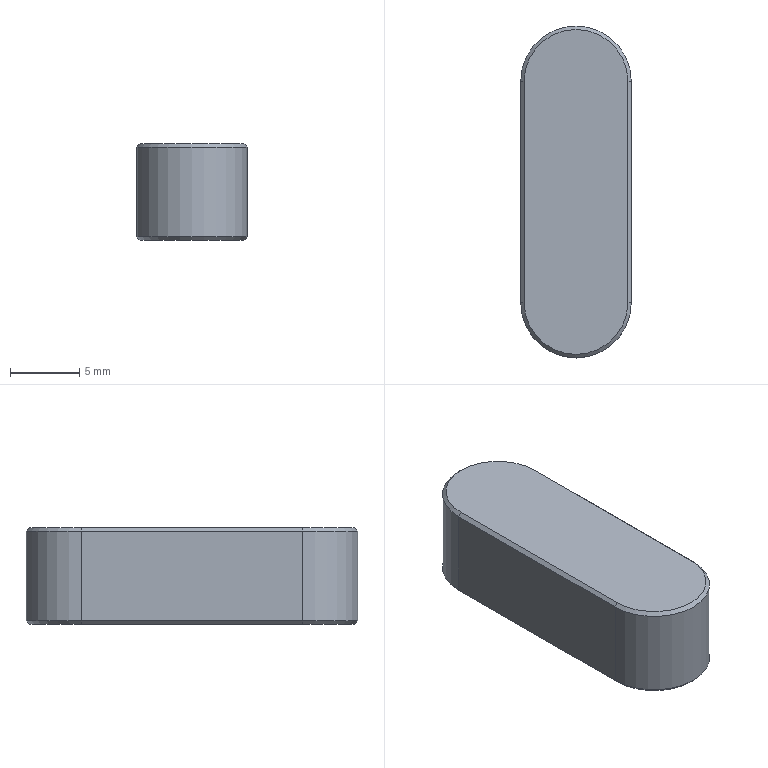Component | NX | KEY_A_8X7X24 | 1 solid | 14 faces | box 8 x 24 x 7 mm | volume 1244 mm3 | plane 8 | cone 4 | cylinder 2 | commonest cylinder face diameters 8 x2
STEP:
#1=CARTESIAN_POINT('',(0.,0.,0.));
#2=DIRECTION('',(0.,0.,1.));
#3=DIRECTION('',(1.,0.,0.));
#4=AXIS2_PLACEMENT_3D('',#1,#2,#3);
#5=CARTESIAN_POINT('',(375.053,-142.75,-118.));
#6=VERTEX_POINT('',#5);
#7=CARTESIAN_POINT('',(375.053,-158.75,-118.));
#8=VERTEX_POINT('',#7);
#9=CARTESIAN_POINT('',(375.053,-150.75,-118.));
#10=DIRECTION('',(0.,-1.,0.));
#11=VECTOR('',#10,1.);
#12=LINE('',#9,#11);
#13=CARTESIAN_POINT('',(378.803,-150.75,-118.));
#14=DIRECTION('',(0.,0.,1.));
#15=DIRECTION('',(1.,0.,0.));
#16=AXIS2_PLACEMENT_3D('',#13,#14,#15);
#17=PLANE('',#16);
#18=CARTESIAN_POINT('',(-3.75,0.));
#19=DIRECTION('',(0.,-1.));
#20=VECTOR('',#19,1.);
#21=LINE('',#18,#20);
#22=(GEOMETRIC_REPRESENTATION_CONTEXT(2)PARAMETRIC_REPRESENTATION_CONTEXT()REPRESENTATION_CONTEXT('',''));
#23=DEFINITIONAL_REPRESENTATION('',(#21),#22);
#24=PCURVE('',#17,#23);
#25=CARTESIAN_POINT('',(374.803,-150.75,-118.25));
#26=DIRECTION('',(0.7071,0.,-0.7071));
#27=DIRECTION('',(0.,1.,0.));
#28=AXIS2_PLACEMENT_3D('',#25,#26,#27);
#29=PLANE('',#28);
#30=CARTESIAN_POINT('',(0.,0.3536));
#31=DIRECTION('',(-1.,0.));
#32=VECTOR('',#31,1.);
#33=LINE('',#30,#32);
#34=(GEOMETRIC_REPRESENTATION_CONTEXT(2)PARAMETRIC_REPRESENTATION_CONTEXT()REPRESENTATION_CONTEXT('',''));
#35=DEFINITIONAL_REPRESENTATION('',(#33),#34);
#36=PCURVE('',#29,#35);
#37=SURFACE_CURVE('',#12,(#24,#36),.PCURVE_S1.);
#38=EDGE_CURVE('',#6,#8,#37,.T.);
#39=ORIENTED_EDGE('',*,*,#38,.T.);
#40=CARTESIAN_POINT('',(382.553,-158.75,-118.));
#41=VERTEX_POINT('',#40);
#42=CARTESIAN_POINT('',(378.803,-158.75,-118.));
#43=DIRECTION('',(0.,0.,1.));
#44=DIRECTION('',(1.,0.,0.));
#45=AXIS2_PLACEMENT_3D('',#42,#43,#44);
#46=CIRCLE('',#45,3.75);
#47=CARTESIAN_POINT('',(0.,-8.));
#48=DIRECTION('',(1.,0.));
#49=AXIS2_PLACEMENT_2D('',#47,#48);
#50=CIRCLE('',#49,3.75);
#51=(GEOMETRIC_REPRESENTATION_CONTEXT(2)PARAMETRIC_REPRESENTATION_CONTEXT()REPRESENTATION_CONTEXT('',''));
#52=DEFINITIONAL_REPRESENTATION('',(#50),#51);
#53=PCURVE('',#17,#52);
#54=CARTESIAN_POINT('',(378.803,-158.75,-118.));
#55=DIRECTION('',(0.,0.,-1.));
#56=DIRECTION('',(-1.,0.,0.));
#57=AXIS2_PLACEMENT_3D('',#54,#55,#56);
#58=CONICAL_SURFACE('',#57,3.75,0.7854);
#59=CARTESIAN_POINT('',(9.425,0.));
#60=DIRECTION('',(-1.,0.));
#61=VECTOR('',#60,1.);
#62=LINE('',#59,#61);
#63=(GEOMETRIC_REPRESENTATION_CONTEXT(2)PARAMETRIC_REPRESENTATION_CONTEXT()REPRESENTATION_CONTEXT('',''));
#64=DEFINITIONAL_REPRESENTATION('',(#62),#63);
#65=PCURVE('',#58,#64);
#66=SURFACE_CURVE('',#46,(#53,#65),.PCURVE_S1.);
#67=EDGE_CURVE('',#8,#41,#66,.T.);
#68=ORIENTED_EDGE('',*,*,#67,.T.);
#69=CARTESIAN_POINT('',(382.553,-142.75,-118.));
#70=VERTEX_POINT('',#69);
#71=CARTESIAN_POINT('',(382.553,-150.75,-118.));
#72=DIRECTION('',(0.,1.,0.));
#73=VECTOR('',#72,1.);
#74=LINE('',#71,#73);
#75=CARTESIAN_POINT('',(3.75,0.));
#76=DIRECTION('',(0.,1.));
#77=VECTOR('',#76,1.);
#78=LINE('',#75,#77);
#79=(GEOMETRIC_REPRESENTATION_CONTEXT(2)PARAMETRIC_REPRESENTATION_CONTEXT()REPRESENTATION_CONTEXT('',''));
#80=DEFINITIONAL_REPRESENTATION('',(#78),#79);
#81=PCURVE('',#17,#80);
#82=CARTESIAN_POINT('',(382.803,-150.75,-118.25));
#83=DIRECTION('',(-0.7071,0.,-0.7071));
#84=DIRECTION('',(0.,-1.,0.));
#85=AXIS2_PLACEMENT_3D('',#82,#83,#84);
#86=PLANE('',#85);
#87=CARTESIAN_POINT('',(0.,0.3536));
#88=DIRECTION('',(-1.,0.));
#89=VECTOR('',#88,1.);
#90=LINE('',#87,#89);
#91=(GEOMETRIC_REPRESENTATION_CONTEXT(2)PARAMETRIC_REPRESENTATION_CONTEXT()REPRESENTATION_CONTEXT('',''));
#92=DEFINITIONAL_REPRESENTATION('',(#90),#91);
#93=PCURVE('',#86,#92);
#94=SURFACE_CURVE('',#74,(#81,#93),.PCURVE_S1.);
#95=EDGE_CURVE('',#41,#70,#94,.T.);
#96=ORIENTED_EDGE('',*,*,#95,.T.);
#97=CARTESIAN_POINT('',(378.803,-142.75,-118.));
#98=DIRECTION('',(0.,0.,1.));
#99=DIRECTION('',(1.,0.,0.));
#100=AXIS2_PLACEMENT_3D('',#97,#98,#99);
#101=CIRCLE('',#100,3.75);
#102=CARTESIAN_POINT('',(0.,8.));
#103=DIRECTION('',(1.,0.));
#104=AXIS2_PLACEMENT_2D('',#102,#103);
#105=CIRCLE('',#104,3.75);
#106=(GEOMETRIC_REPRESENTATION_CONTEXT(2)PARAMETRIC_REPRESENTATION_CONTEXT()REPRESENTATION_CONTEXT('',''));
#107=DEFINITIONAL_REPRESENTATION('',(#105),#106);
#108=PCURVE('',#17,#107);
#109=CARTESIAN_POINT('',(378.803,-142.75,-118.));
#110=DIRECTION('',(0.,0.,-1.));
#111=DIRECTION('',(-1.,0.,0.));
#112=AXIS2_PLACEMENT_3D('',#109,#110,#111);
#113=CONICAL_SURFACE('',#112,3.75,0.7854);
#114=CARTESIAN_POINT('',(3.142,0.));
#115=DIRECTION('',(-1.,0.));
#116=VECTOR('',#115,1.);
#117=LINE('',#114,#116);
#118=(GEOMETRIC_REPRESENTATION_CONTEXT(2)PARAMETRIC_REPRESENTATION_CONTEXT()REPRESENTATION_CONTEXT('',''));
#119=DEFINITIONAL_REPRESENTATION('',(#117),#118);
#120=PCURVE('',#113,#119);
#121=SURFACE_CURVE('',#101,(#108,#120),.PCURVE_S1.);
#122=EDGE_CURVE('',#70,#6,#121,.T.);
#123=ORIENTED_EDGE('',*,*,#122,.T.);
#124=EDGE_LOOP('',(#39,#68,#96,#123));
#125=FACE_BOUND('',#124,.T.);
#126=ADVANCED_FACE('',(#125),#17,.T.);
#127=CARTESIAN_POINT('',(374.803,-142.75,-118.25));
#128=VERTEX_POINT('',#127);
#129=CARTESIAN_POINT('',(374.803,-142.75,-124.75));
#130=VERTEX_POINT('',#129);
#131=CARTESIAN_POINT('',(374.803,-142.75,-125.));
#132=DIRECTION('',(0.,0.,-1.));
#133=VECTOR('',#132,1.);
#134=LINE('',#131,#133);
#135=CARTESIAN_POINT('',(374.803,-150.75,-125.));
#136=DIRECTION('',(-1.,0.,0.));
#137=DIRECTION('',(0.,0.,1.));
#138=AXIS2_PLACEMENT_3D('',#135,#136,#137);
#139=PLANE('',#138);
#140=CARTESIAN_POINT('',(0.,8.));
#141=DIRECTION('',(-1.,0.));
#142=VECTOR('',#141,1.);
#143=LINE('',#140,#142);
#144=(GEOMETRIC_REPRESENTATION_CONTEXT(2)PARAMETRIC_REPRESENTATION_CONTEXT()REPRESENTATION_CONTEXT('',''));
#145=DEFINITIONAL_REPRESENTATION('',(#143),#144);
#146=PCURVE('',#139,#145);
#147=CARTESIAN_POINT('',(378.803,-142.75,-125.));
#148=DIRECTION('',(0.,0.,1.));
#149=DIRECTION('',(1.,0.,0.));
#150=AXIS2_PLACEMENT_3D('',#147,#148,#149);
#151=CYLINDRICAL_SURFACE('',#150,4.);
#152=CARTESIAN_POINT('',(3.142,0.));
#153=DIRECTION('',(0.,-1.));
#154=VECTOR('',#153,1.);
#155=LINE('',#152,#154);
#156=(GEOMETRIC_REPRESENTATION_CONTEXT(2)PARAMETRIC_REPRESENTATION_CONTEXT()REPRESENTATION_CONTEXT('',''));
#157=DEFINITIONAL_REPRESENTATION('',(#155),#156);
#158=PCURVE('',#151,#157);
#159=SURFACE_CURVE('',#134,(#146,#158),.PCURVE_S1.);
#160=EDGE_CURVE('',#128,#130,#159,.T.);
#161=ORIENTED_EDGE('',*,*,#160,.T.);
#162=CARTESIAN_POINT('',(374.803,-158.75,-124.75));
#163=VERTEX_POINT('',#162);
#164=CARTESIAN_POINT('',(374.803,-150.75,-124.75));
#165=DIRECTION('',(0.,-1.,0.));
#166=VECTOR('',#165,1.);
#167=LINE('',#164,#166);
#168=CARTESIAN_POINT('',(0.25,0.));
#169=DIRECTION('',(0.,-1.));
#170=VECTOR('',#169,1.);
#171=LINE('',#168,#170);
#172=(GEOMETRIC_REPRESENTATION_CONTEXT(2)PARAMETRIC_REPRESENTATION_CONTEXT()REPRESENTATION_CONTEXT('',''));
#173=DEFINITIONAL_REPRESENTATION('',(#171),#172);
#174=PCURVE('',#139,#173);
#175=CARTESIAN_POINT('',(374.803,-150.75,-124.75));
#176=DIRECTION('',(0.7071,0.,0.7071));
#177=DIRECTION('',(0.,-1.,0.));
#178=AXIS2_PLACEMENT_3D('',#175,#176,#177);
#179=PLANE('',#178);
#180=CARTESIAN_POINT('',(0.,0.));
#181=DIRECTION('',(1.,0.));
#182=VECTOR('',#181,1.);
#183=LINE('',#180,#182);
#184=(GEOMETRIC_REPRESENTATION_CONTEXT(2)PARAMETRIC_REPRESENTATION_CONTEXT()REPRESENTATION_CONTEXT('',''));
#185=DEFINITIONAL_REPRESENTATION('',(#183),#184);
#186=PCURVE('',#179,#185);
#187=SURFACE_CURVE('',#167,(#174,#186),.PCURVE_S1.);
#188=EDGE_CURVE('',#130,#163,#187,.T.);
#189=ORIENTED_EDGE('',*,*,#188,.T.);
#190=CARTESIAN_POINT('',(374.803,-158.75,-118.25));
#191=VERTEX_POINT('',#190);
#192=CARTESIAN_POINT('',(374.803,-158.75,-125.));
#193=DIRECTION('',(0.,0.,1.));
#194=VECTOR('',#193,1.);
#195=LINE('',#192,#194);
#196=CARTESIAN_POINT('',(0.,-8.));
#197=DIRECTION('',(1.,0.));
#198=VECTOR('',#197,1.);
#199=LINE('',#196,#198);
#200=(GEOMETRIC_REPRESENTATION_CONTEXT(2)PARAMETRIC_REPRESENTATION_CONTEXT()REPRESENTATION_CONTEXT('',''));
#201=DEFINITIONAL_REPRESENTATION('',(#199),#200);
#202=PCURVE('',#139,#201);
#203=CARTESIAN_POINT('',(378.803,-158.75,-125.));
#204=DIRECTION('',(0.,0.,1.));
#205=DIRECTION('',(1.,0.,0.));
#206=AXIS2_PLACEMENT_3D('',#203,#204,#205);
#207=CYLINDRICAL_SURFACE('',#206,4.);
#208=CARTESIAN_POINT('',(3.142,0.));
#209=DIRECTION('',(0.,1.));
#210=VECTOR('',#209,1.);
#211=LINE('',#208,#210);
#212=(GEOMETRIC_REPRESENTATION_CONTEXT(2)PARAMETRIC_REPRESENTATION_CONTEXT()REPRESENTATION_CONTEXT('',''));
#213=DEFINITIONAL_REPRESENTATION('',(#211),#212);
#214=PCURVE('',#207,#213);
#215=SURFACE_CURVE('',#195,(#202,#214),.PCURVE_S1.);
#216=EDGE_CURVE('',#163,#191,#215,.T.);
#217=ORIENTED_EDGE('',*,*,#216,.T.);
#218=CARTESIAN_POINT('',(374.803,-150.75,-118.25));
#219=DIRECTION('',(0.,1.,0.));
#220=VECTOR('',#219,1.);
#221=LINE('',#218,#220);
#222=CARTESIAN_POINT('',(6.75,0.));
#223=DIRECTION('',(0.,1.));
#224=VECTOR('',#223,1.);
#225=LINE('',#222,#224);
#226=(GEOMETRIC_REPRESENTATION_CONTEXT(2)PARAMETRIC_REPRESENTATION_CONTEXT()REPRESENTATION_CONTEXT('',''));
#227=DEFINITIONAL_REPRESENTATION('',(#225),#226);
#228=PCURVE('',#139,#227);
#229=CARTESIAN_POINT('',(0.,0.));
#230=DIRECTION('',(1.,0.));
#231=VECTOR('',#230,1.);
#232=LINE('',#229,#231);
#233=(GEOMETRIC_REPRESENTATION_CONTEXT(2)PARAMETRIC_REPRESENTATION_CONTEXT()REPRESENTATION_CONTEXT('',''));
#234=DEFINITIONAL_REPRESENTATION('',(#232),#233);
#235=PCURVE('',#29,#234);
#236=SURFACE_CURVE('',#221,(#228,#235),.PCURVE_S1.);
#237=EDGE_CURVE('',#191,#128,#236,.T.);
#238=ORIENTED_EDGE('',*,*,#237,.T.);
#239=EDGE_LOOP('',(#161,#189,#217,#238));
#240=FACE_BOUND('',#239,.T.);
#241=ADVANCED_FACE('',(#240),#139,.T.);
#242=CARTESIAN_POINT('',(382.553,-142.75,-125.));
#243=VERTEX_POINT('',#242);
#244=CARTESIAN_POINT('',(382.553,-158.75,-125.));
#245=VERTEX_POINT('',#244);
#246=CARTESIAN_POINT('',(382.553,-150.75,-125.));
#247=DIRECTION('',(0.,-1.,0.));
#248=VECTOR('',#247,1.);
#249=LINE('',#246,#248);
#250=CARTESIAN_POINT('',(378.803,-150.75,-125.));
#251=DIRECTION('',(0.,0.,-1.));
#252=DIRECTION('',(-1.,0.,0.));
#253=AXIS2_PLACEMENT_3D('',#250,#251,#252);
#254=PLANE('',#253);
#255=CARTESIAN_POINT('',(-3.75,0.));
#256=DIRECTION('',(0.,-1.));
#257=VECTOR('',#256,1.);
#258=LINE('',#255,#257);
#259=(GEOMETRIC_REPRESENTATION_CONTEXT(2)PARAMETRIC_REPRESENTATION_CONTEXT()REPRESENTATION_CONTEXT('',''));
#260=DEFINITIONAL_REPRESENTATION('',(#258),#259);
#261=PCURVE('',#254,#260);
#262=CARTESIAN_POINT('',(382.803,-150.75,-124.75));
#263=DIRECTION('',(-0.7071,0.,0.7071));
#264=DIRECTION('',(0.,1.,0.));
#265=AXIS2_PLACEMENT_3D('',#262,#263,#264);
#266=PLANE('',#265);
#267=CARTESIAN_POINT('',(0.,0.3536));
#268=DIRECTION('',(-1.,0.));
#269=VECTOR('',#268,1.);
#270=LINE('',#267,#269);
#271=(GEOMETRIC_REPRESENTATION_CONTEXT(2)PARAMETRIC_REPRESENTATION_CONTEXT()REPRESENTATION_CONTEXT('',''));
#272=DEFINITIONAL_REPRESENTATION('',(#270),#271);
#273=PCURVE('',#266,#272);
#274=SURFACE_CURVE('',#249,(#261,#273),.PCURVE_S1.);
#275=EDGE_CURVE('',#243,#245,#274,.T.);
#276=ORIENTED_EDGE('',*,*,#275,.T.);
#277=CARTESIAN_POINT('',(375.053,-158.75,-125.));
#278=VERTEX_POINT('',#277);
#279=CARTESIAN_POINT('',(378.803,-158.75,-125.));
#280=DIRECTION('',(0.,0.,-1.));
#281=DIRECTION('',(-1.,0.,0.));
#282=AXIS2_PLACEMENT_3D('',#279,#280,#281);
#283=CIRCLE('',#282,3.75);
#284=CARTESIAN_POINT('',(0.,-8.));
#285=DIRECTION('',(1.,0.));
#286=AXIS2_PLACEMENT_2D('',#284,#285);
#287=CIRCLE('',#286,3.75);
#288=(GEOMETRIC_REPRESENTATION_CONTEXT(2)PARAMETRIC_REPRESENTATION_CONTEXT()REPRESENTATION_CONTEXT('',''));
#289=DEFINITIONAL_REPRESENTATION('',(#287),#288);
#290=PCURVE('',#254,#289);
#291=CARTESIAN_POINT('',(378.803,-158.75,-125.));
#292=DIRECTION('',(0.,0.,1.));
#293=DIRECTION('',(1.,0.,0.));
#294=AXIS2_PLACEMENT_3D('',#291,#292,#293);
#295=CONICAL_SURFACE('',#294,3.75,0.7854);
#296=CARTESIAN_POINT('',(9.425,0.));
#297=DIRECTION('',(-1.,0.));
#298=VECTOR('',#297,1.);
#299=LINE('',#296,#298);
#300=(GEOMETRIC_REPRESENTATION_CONTEXT(2)PARAMETRIC_REPRESENTATION_CONTEXT()REPRESENTATION_CONTEXT('',''));
#301=DEFINITIONAL_REPRESENTATION('',(#299),#300);
#302=PCURVE('',#295,#301);
#303=SURFACE_CURVE('',#283,(#290,#302),.PCURVE_S1.);
#304=EDGE_CURVE('',#245,#278,#303,.T.);
#305=ORIENTED_EDGE('',*,*,#304,.T.);
#306=CARTESIAN_POINT('',(375.053,-142.75,-125.));
#307=VERTEX_POINT('',#306);
#308=CARTESIAN_POINT('',(375.053,-150.75,-125.));
#309=DIRECTION('',(0.,1.,0.));
#310=VECTOR('',#309,1.);
#311=LINE('',#308,#310);
#312=CARTESIAN_POINT('',(3.75,0.));
#313=DIRECTION('',(0.,1.));
#314=VECTOR('',#313,1.);
#315=LINE('',#312,#314);
#316=(GEOMETRIC_REPRESENTATION_CONTEXT(2)PARAMETRIC_REPRESENTATION_CONTEXT()REPRESENTATION_CONTEXT('',''));
#317=DEFINITIONAL_REPRESENTATION('',(#315),#316);
#318=PCURVE('',#254,#317);
#319=CARTESIAN_POINT('',(0.,0.3536));
#320=DIRECTION('',(-1.,0.));
#321=VECTOR('',#320,1.);
#322=LINE('',#319,#321);
#323=(GEOMETRIC_REPRESENTATION_CONTEXT(2)PARAMETRIC_REPRESENTATION_CONTEXT()REPRESENTATION_CONTEXT('',''));
#324=DEFINITIONAL_REPRESENTATION('',(#322),#323);
#325=PCURVE('',#179,#324);
#326=SURFACE_CURVE('',#311,(#318,#325),.PCURVE_S1.);
#327=EDGE_CURVE('',#278,#307,#326,.T.);
#328=ORIENTED_EDGE('',*,*,#327,.T.);
#329=CARTESIAN_POINT('',(378.803,-142.75,-125.));
#330=DIRECTION('',(0.,0.,-1.));
#331=DIRECTION('',(-1.,0.,0.));
#332=AXIS2_PLACEMENT_3D('',#329,#330,#331);
#333=CIRCLE('',#332,3.75);
#334=CARTESIAN_POINT('',(0.,8.));
#335=DIRECTION('',(1.,0.));
#336=AXIS2_PLACEMENT_2D('',#334,#335);
#337=CIRCLE('',#336,3.75);
#338=(GEOMETRIC_REPRESENTATION_CONTEXT(2)PARAMETRIC_REPRESENTATION_CONTEXT()REPRESENTATION_CONTEXT('',''));
#339=DEFINITIONAL_REPRESENTATION('',(#337),#338);
#340=PCURVE('',#254,#339);
#341=CARTESIAN_POINT('',(378.803,-142.75,-125.));
#342=DIRECTION('',(0.,0.,1.));
#343=DIRECTION('',(1.,0.,0.));
#344=AXIS2_PLACEMENT_3D('',#341,#342,#343);
#345=CONICAL_SURFACE('',#344,3.75,0.7854);
#346=CARTESIAN_POINT('',(3.142,0.));
#347=DIRECTION('',(-1.,0.));
#348=VECTOR('',#347,1.);
#349=LINE('',#346,#348);
#350=(GEOMETRIC_REPRESENTATION_CONTEXT(2)PARAMETRIC_REPRESENTATION_CONTEXT()REPRESENTATION_CONTEXT('',''));
#351=DEFINITIONAL_REPRESENTATION('',(#349),#350);
#352=PCURVE('',#345,#351);
#353=SURFACE_CURVE('',#333,(#340,#352),.PCURVE_S1.);
#354=EDGE_CURVE('',#307,#243,#353,.T.);
#355=ORIENTED_EDGE('',*,*,#354,.T.);
#356=EDGE_LOOP('',(#276,#305,#328,#355));
#357=FACE_BOUND('',#356,.T.);
#358=ADVANCED_FACE('',(#357),#254,.T.);
#359=CARTESIAN_POINT('',(382.803,-158.75,-118.25));
#360=VERTEX_POINT('',#359);
#361=CARTESIAN_POINT('',(382.803,-158.75,-124.75));
#362=VERTEX_POINT('',#361);
#363=CARTESIAN_POINT('',(382.803,-158.75,-125.));
#364=DIRECTION('',(0.,0.,-1.));
#365=VECTOR('',#364,1.);
#366=LINE('',#363,#365);
#367=CARTESIAN_POINT('',(382.803,-150.75,-125.));
#368=DIRECTION('',(1.,0.,0.));
#369=DIRECTION('',(0.,0.,-1.));
#370=AXIS2_PLACEMENT_3D('',#367,#368,#369);
#371=PLANE('',#370);
#372=CARTESIAN_POINT('',(0.,-8.));
#373=DIRECTION('',(1.,0.));
#374=VECTOR('',#373,1.);
#375=LINE('',#372,#374);
#376=(GEOMETRIC_REPRESENTATION_CONTEXT(2)PARAMETRIC_REPRESENTATION_CONTEXT()REPRESENTATION_CONTEXT('',''));
#377=DEFINITIONAL_REPRESENTATION('',(#375),#376);
#378=PCURVE('',#371,#377);
#379=CARTESIAN_POINT('',(6.283,0.));
#380=DIRECTION('',(0.,-1.));
#381=VECTOR('',#380,1.);
#382=LINE('',#379,#381);
#383=(GEOMETRIC_REPRESENTATION_CONTEXT(2)PARAMETRIC_REPRESENTATION_CONTEXT()REPRESENTATION_CONTEXT('',''));
#384=DEFINITIONAL_REPRESENTATION('',(#382),#383);
#385=PCURVE('',#207,#384);
#386=SURFACE_CURVE('',#366,(#378,#385),.PCURVE_S1.);
#387=EDGE_CURVE('',#360,#362,#386,.T.);
#388=ORIENTED_EDGE('',*,*,#387,.T.);
#389=CARTESIAN_POINT('',(382.803,-142.75,-124.75));
#390=VERTEX_POINT('',#389);
#391=CARTESIAN_POINT('',(382.803,-150.75,-124.75));
#392=DIRECTION('',(0.,1.,0.));
#393=VECTOR('',#392,1.);
#394=LINE('',#391,#393);
#395=CARTESIAN_POINT('',(-0.25,0.));
#396=DIRECTION('',(0.,1.));
#397=VECTOR('',#396,1.);
#398=LINE('',#395,#397);
#399=(GEOMETRIC_REPRESENTATION_CONTEXT(2)PARAMETRIC_REPRESENTATION_CONTEXT()REPRESENTATION_CONTEXT('',''));
#400=DEFINITIONAL_REPRESENTATION('',(#398),#399);
#401=PCURVE('',#371,#400);
#402=CARTESIAN_POINT('',(0.,0.));
#403=DIRECTION('',(1.,0.));
#404=VECTOR('',#403,1.);
#405=LINE('',#402,#404);
#406=(GEOMETRIC_REPRESENTATION_CONTEXT(2)PARAMETRIC_REPRESENTATION_CONTEXT()REPRESENTATION_CONTEXT('',''));
#407=DEFINITIONAL_REPRESENTATION('',(#405),#406);
#408=PCURVE('',#266,#407);
#409=SURFACE_CURVE('',#394,(#401,#408),.PCURVE_S1.);
#410=EDGE_CURVE('',#362,#390,#409,.T.);
#411=ORIENTED_EDGE('',*,*,#410,.T.);
#412=CARTESIAN_POINT('',(382.803,-142.75,-118.25));
#413=VERTEX_POINT('',#412);
#414=CARTESIAN_POINT('',(382.803,-142.75,-125.));
#415=DIRECTION('',(0.,0.,1.));
#416=VECTOR('',#415,1.);
#417=LINE('',#414,#416);
#418=CARTESIAN_POINT('',(0.,8.));
#419=DIRECTION('',(-1.,0.));
#420=VECTOR('',#419,1.);
#421=LINE('',#418,#420);
#422=(GEOMETRIC_REPRESENTATION_CONTEXT(2)PARAMETRIC_REPRESENTATION_CONTEXT()REPRESENTATION_CONTEXT('',''));
#423=DEFINITIONAL_REPRESENTATION('',(#421),#422);
#424=PCURVE('',#371,#423);
#425=CARTESIAN_POINT('',(0.,0.));
#426=DIRECTION('',(0.,1.));
#427=VECTOR('',#426,1.);
#428=LINE('',#425,#427);
#429=(GEOMETRIC_REPRESENTATION_CONTEXT(2)PARAMETRIC_REPRESENTATION_CONTEXT()REPRESENTATION_CONTEXT('',''));
#430=DEFINITIONAL_REPRESENTATION('',(#428),#429);
#431=PCURVE('',#151,#430);
#432=SURFACE_CURVE('',#417,(#424,#431),.PCURVE_S1.);
#433=EDGE_CURVE('',#390,#413,#432,.T.);
#434=ORIENTED_EDGE('',*,*,#433,.T.);
#435=CARTESIAN_POINT('',(382.803,-150.75,-118.25));
#436=DIRECTION('',(0.,-1.,0.));
#437=VECTOR('',#436,1.);
#438=LINE('',#435,#437);
#439=CARTESIAN_POINT('',(-6.75,0.));
#440=DIRECTION('',(0.,-1.));
#441=VECTOR('',#440,1.);
#442=LINE('',#439,#441);
#443=(GEOMETRIC_REPRESENTATION_CONTEXT(2)PARAMETRIC_REPRESENTATION_CONTEXT()REPRESENTATION_CONTEXT('',''));
#444=DEFINITIONAL_REPRESENTATION('',(#442),#443);
#445=PCURVE('',#371,#444);
#446=CARTESIAN_POINT('',(0.,0.));
#447=DIRECTION('',(1.,0.));
#448=VECTOR('',#447,1.);
#449=LINE('',#446,#448);
#450=(GEOMETRIC_REPRESENTATION_CONTEXT(2)PARAMETRIC_REPRESENTATION_CONTEXT()REPRESENTATION_CONTEXT('',''));
#451=DEFINITIONAL_REPRESENTATION('',(#449),#450);
#452=PCURVE('',#86,#451);
#453=SURFACE_CURVE('',#438,(#445,#452),.PCURVE_S1.);
#454=EDGE_CURVE('',#413,#360,#453,.T.);
#455=ORIENTED_EDGE('',*,*,#454,.T.);
#456=EDGE_LOOP('',(#388,#411,#434,#455));
#457=FACE_BOUND('',#456,.T.);
#458=ADVANCED_FACE('',(#457),#371,.T.);
#459=ORIENTED_EDGE('',*,*,#433,.F.);
#460=CARTESIAN_POINT('',(378.803,-142.75,-124.75));
#461=DIRECTION('',(0.,0.,1.));
#462=DIRECTION('',(-1.,0.,0.));
#463=AXIS2_PLACEMENT_3D('',#460,#461,#462);
#464=CIRCLE('',#463,4.);
#465=CARTESIAN_POINT('',(-3.142,0.25));
#466=DIRECTION('',(1.,0.));
#467=VECTOR('',#466,1.);
#468=LINE('',#465,#467);
#469=(GEOMETRIC_REPRESENTATION_CONTEXT(2)PARAMETRIC_REPRESENTATION_CONTEXT()REPRESENTATION_CONTEXT('',''));
#470=DEFINITIONAL_REPRESENTATION('',(#468),#469);
#471=PCURVE('',#151,#470);
#472=CARTESIAN_POINT('',(-3.142,0.25));
#473=DIRECTION('',(1.,0.));
#474=VECTOR('',#473,1.);
#475=LINE('',#472,#474);
#476=(GEOMETRIC_REPRESENTATION_CONTEXT(2)PARAMETRIC_REPRESENTATION_CONTEXT()REPRESENTATION_CONTEXT('',''));
#477=DEFINITIONAL_REPRESENTATION('',(#475),#476);
#478=PCURVE('',#345,#477);
#479=SURFACE_CURVE('',#464,(#471,#478),.PCURVE_S1.);
#480=EDGE_CURVE('',#390,#130,#479,.T.);
#481=ORIENTED_EDGE('',*,*,#480,.T.);
#482=ORIENTED_EDGE('',*,*,#160,.F.);
#483=CARTESIAN_POINT('',(378.803,-142.75,-118.25));
#484=DIRECTION('',(0.,0.,-1.));
#485=DIRECTION('',(1.,0.,0.));
#486=AXIS2_PLACEMENT_3D('',#483,#484,#485);
#487=CIRCLE('',#486,4.);
#488=CARTESIAN_POINT('',(6.283,6.75));
#489=DIRECTION('',(-1.,0.));
#490=VECTOR('',#489,1.);
#491=LINE('',#488,#490);
#492=(GEOMETRIC_REPRESENTATION_CONTEXT(2)PARAMETRIC_REPRESENTATION_CONTEXT()REPRESENTATION_CONTEXT('',''));
#493=DEFINITIONAL_REPRESENTATION('',(#491),#492);
#494=PCURVE('',#151,#493);
#495=CARTESIAN_POINT('',(-3.142,0.25));
#496=DIRECTION('',(1.,0.));
#497=VECTOR('',#496,1.);
#498=LINE('',#495,#497);
#499=(GEOMETRIC_REPRESENTATION_CONTEXT(2)PARAMETRIC_REPRESENTATION_CONTEXT()REPRESENTATION_CONTEXT('',''));
#500=DEFINITIONAL_REPRESENTATION('',(#498),#499);
#501=PCURVE('',#113,#500);
#502=SURFACE_CURVE('',#487,(#494,#501),.PCURVE_S1.);
#503=EDGE_CURVE('',#128,#413,#502,.T.);
#504=ORIENTED_EDGE('',*,*,#503,.T.);
#505=EDGE_LOOP('',(#459,#481,#482,#504));
#506=FACE_BOUND('',#505,.T.);
#507=ADVANCED_FACE('',(#506),#151,.T.);
#508=ORIENTED_EDGE('',*,*,#216,.F.);
#509=CARTESIAN_POINT('',(378.803,-158.75,-124.75));
#510=DIRECTION('',(0.,0.,1.));
#511=DIRECTION('',(-1.,0.,0.));
#512=AXIS2_PLACEMENT_3D('',#509,#510,#511);
#513=CIRCLE('',#512,4.);
#514=CARTESIAN_POINT('',(3.142,0.25));
#515=DIRECTION('',(1.,0.));
#516=VECTOR('',#515,1.);
#517=LINE('',#514,#516);
#518=(GEOMETRIC_REPRESENTATION_CONTEXT(2)PARAMETRIC_REPRESENTATION_CONTEXT()REPRESENTATION_CONTEXT('',''));
#519=DEFINITIONAL_REPRESENTATION('',(#517),#518);
#520=PCURVE('',#207,#519);
#521=CARTESIAN_POINT('',(3.142,0.25));
#522=DIRECTION('',(1.,0.));
#523=VECTOR('',#522,1.);
#524=LINE('',#521,#523);
#525=(GEOMETRIC_REPRESENTATION_CONTEXT(2)PARAMETRIC_REPRESENTATION_CONTEXT()REPRESENTATION_CONTEXT('',''));
#526=DEFINITIONAL_REPRESENTATION('',(#524),#525);
#527=PCURVE('',#295,#526);
#528=SURFACE_CURVE('',#513,(#520,#527),.PCURVE_S1.);
#529=EDGE_CURVE('',#163,#362,#528,.T.);
#530=ORIENTED_EDGE('',*,*,#529,.T.);
#531=ORIENTED_EDGE('',*,*,#387,.F.);
#532=CARTESIAN_POINT('',(378.803,-158.75,-118.25));
#533=DIRECTION('',(0.,0.,-1.));
#534=DIRECTION('',(1.,0.,0.));
#535=AXIS2_PLACEMENT_3D('',#532,#533,#534);
#536=CIRCLE('',#535,4.);
#537=CARTESIAN_POINT('',(6.283,6.75));
#538=DIRECTION('',(-1.,0.));
#539=VECTOR('',#538,1.);
#540=LINE('',#537,#539);
#541=(GEOMETRIC_REPRESENTATION_CONTEXT(2)PARAMETRIC_REPRESENTATION_CONTEXT()REPRESENTATION_CONTEXT('',''));
#542=DEFINITIONAL_REPRESENTATION('',(#540),#541);
#543=PCURVE('',#207,#542);
#544=CARTESIAN_POINT('',(3.142,0.25));
#545=DIRECTION('',(1.,0.));
#546=VECTOR('',#545,1.);
#547=LINE('',#544,#546);
#548=(GEOMETRIC_REPRESENTATION_CONTEXT(2)PARAMETRIC_REPRESENTATION_CONTEXT()REPRESENTATION_CONTEXT('',''));
#549=DEFINITIONAL_REPRESENTATION('',(#547),#548);
#550=PCURVE('',#58,#549);
#551=SURFACE_CURVE('',#536,(#543,#550),.PCURVE_S1.);
#552=EDGE_CURVE('',#360,#191,#551,.T.);
#553=ORIENTED_EDGE('',*,*,#552,.T.);
#554=EDGE_LOOP('',(#508,#530,#531,#553));
#555=FACE_BOUND('',#554,.T.);
#556=ADVANCED_FACE('',(#555),#207,.T.);
#557=CARTESIAN_POINT('',(374.803,-142.75,-124.75));
#558=DIRECTION('',(0.7071,0.,-0.7071));
#559=VECTOR('',#558,1.);
#560=LINE('',#557,#559);
#561=CARTESIAN_POINT('',(3.142,0.25));
#562=DIRECTION('',(0.,-1.));
#563=VECTOR('',#562,1.);
#564=LINE('',#561,#563);
#565=(GEOMETRIC_REPRESENTATION_CONTEXT(2)PARAMETRIC_REPRESENTATION_CONTEXT()REPRESENTATION_CONTEXT('',''));
#566=DEFINITIONAL_REPRESENTATION('',(#564),#565);
#567=PCURVE('',#345,#566);
#568=CARTESIAN_POINT('',(-8.,0.));
#569=DIRECTION('',(0.,1.));
#570=VECTOR('',#569,1.);
#571=LINE('',#568,#570);
#572=(GEOMETRIC_REPRESENTATION_CONTEXT(2)PARAMETRIC_REPRESENTATION_CONTEXT()REPRESENTATION_CONTEXT('',''));
#573=DEFINITIONAL_REPRESENTATION('',(#571),#572);
#574=PCURVE('',#179,#573);
#575=SURFACE_CURVE('',#560,(#567,#574),.PCURVE_S1.);
#576=EDGE_CURVE('',#130,#307,#575,.T.);
#577=ORIENTED_EDGE('',*,*,#576,.F.);
#578=ORIENTED_EDGE('',*,*,#480,.F.);
#579=CARTESIAN_POINT('',(382.553,-142.75,-125.));
#580=DIRECTION('',(0.7071,0.,0.7071));
#581=VECTOR('',#580,1.);
#582=LINE('',#579,#581);
#583=CARTESIAN_POINT('',(0.,0.));
#584=DIRECTION('',(0.,1.));
#585=VECTOR('',#584,1.);
#586=LINE('',#583,#585);
#587=(GEOMETRIC_REPRESENTATION_CONTEXT(2)PARAMETRIC_REPRESENTATION_CONTEXT()REPRESENTATION_CONTEXT('',''));
#588=DEFINITIONAL_REPRESENTATION('',(#586),#587);
#589=PCURVE('',#345,#588);
#590=CARTESIAN_POINT('',(8.,0.3536));
#591=DIRECTION('',(0.,-1.));
#592=VECTOR('',#591,1.);
#593=LINE('',#590,#592);
#594=(GEOMETRIC_REPRESENTATION_CONTEXT(2)PARAMETRIC_REPRESENTATION_CONTEXT()REPRESENTATION_CONTEXT('',''));
#595=DEFINITIONAL_REPRESENTATION('',(#593),#594);
#596=PCURVE('',#266,#595);
#597=SURFACE_CURVE('',#582,(#589,#596),.PCURVE_S1.);
#598=EDGE_CURVE('',#243,#390,#597,.T.);
#599=ORIENTED_EDGE('',*,*,#598,.F.);
#600=ORIENTED_EDGE('',*,*,#354,.F.);
#601=EDGE_LOOP('',(#577,#578,#599,#600));
#602=FACE_BOUND('',#601,.T.);
#603=ADVANCED_FACE('',(#602),#345,.T.);
#604=ORIENTED_EDGE('',*,*,#598,.T.);
#605=ORIENTED_EDGE('',*,*,#410,.F.);
#606=CARTESIAN_POINT('',(382.553,-158.75,-125.));
#607=DIRECTION('',(0.7071,0.,0.7071));
#608=VECTOR('',#607,1.);
#609=LINE('',#606,#608);
#610=CARTESIAN_POINT('',(-8.,0.3536));
#611=DIRECTION('',(0.,-1.));
#612=VECTOR('',#611,1.);
#613=LINE('',#610,#612);
#614=(GEOMETRIC_REPRESENTATION_CONTEXT(2)PARAMETRIC_REPRESENTATION_CONTEXT()REPRESENTATION_CONTEXT('',''));
#615=DEFINITIONAL_REPRESENTATION('',(#613),#614);
#616=PCURVE('',#266,#615);
#617=CARTESIAN_POINT('',(6.283,0.));
#618=DIRECTION('',(0.,1.));
#619=VECTOR('',#618,1.);
#620=LINE('',#617,#619);
#621=(GEOMETRIC_REPRESENTATION_CONTEXT(2)PARAMETRIC_REPRESENTATION_CONTEXT()REPRESENTATION_CONTEXT('',''));
#622=DEFINITIONAL_REPRESENTATION('',(#620),#621);
#623=PCURVE('',#295,#622);
#624=SURFACE_CURVE('',#609,(#616,#623),.PCURVE_S1.);
#625=EDGE_CURVE('',#245,#362,#624,.T.);
#626=ORIENTED_EDGE('',*,*,#625,.F.);
#627=ORIENTED_EDGE('',*,*,#275,.F.);
#628=EDGE_LOOP('',(#604,#605,#626,#627));
#629=FACE_BOUND('',#628,.T.);
#630=ADVANCED_FACE('',(#629),#266,.F.);
#631=ORIENTED_EDGE('',*,*,#576,.T.);
#632=ORIENTED_EDGE('',*,*,#327,.F.);
#633=CARTESIAN_POINT('',(374.803,-158.75,-124.75));
#634=DIRECTION('',(0.7071,0.,-0.7071));
#635=VECTOR('',#634,1.);
#636=LINE('',#633,#635);
#637=CARTESIAN_POINT('',(8.,0.));
#638=DIRECTION('',(0.,1.));
#639=VECTOR('',#638,1.);
#640=LINE('',#637,#639);
#641=(GEOMETRIC_REPRESENTATION_CONTEXT(2)PARAMETRIC_REPRESENTATION_CONTEXT()REPRESENTATION_CONTEXT('',''));
#642=DEFINITIONAL_REPRESENTATION('',(#640),#641);
#643=PCURVE('',#179,#642);
#644=CARTESIAN_POINT('',(3.142,0.25));
#645=DIRECTION('',(0.,-1.));
#646=VECTOR('',#645,1.);
#647=LINE('',#644,#646);
#648=(GEOMETRIC_REPRESENTATION_CONTEXT(2)PARAMETRIC_REPRESENTATION_CONTEXT()REPRESENTATION_CONTEXT('',''));
#649=DEFINITIONAL_REPRESENTATION('',(#647),#648);
#650=PCURVE('',#295,#649);
#651=SURFACE_CURVE('',#636,(#643,#650),.PCURVE_S1.);
#652=EDGE_CURVE('',#163,#278,#651,.T.);
#653=ORIENTED_EDGE('',*,*,#652,.F.);
#654=ORIENTED_EDGE('',*,*,#188,.F.);
#655=EDGE_LOOP('',(#631,#632,#653,#654));
#656=FACE_BOUND('',#655,.T.);
#657=ADVANCED_FACE('',(#656),#179,.F.);
#658=ORIENTED_EDGE('',*,*,#625,.T.);
#659=ORIENTED_EDGE('',*,*,#529,.F.);
#660=ORIENTED_EDGE('',*,*,#652,.T.);
#661=ORIENTED_EDGE('',*,*,#304,.F.);
#662=EDGE_LOOP('',(#658,#659,#660,#661));
#663=FACE_BOUND('',#662,.T.);
#664=ADVANCED_FACE('',(#663),#295,.T.);
#665=CARTESIAN_POINT('',(382.803,-142.75,-118.25));
#666=DIRECTION('',(-0.7071,0.,0.7071));
#667=VECTOR('',#666,1.);
#668=LINE('',#665,#667);
#669=CARTESIAN_POINT('',(3.142,0.25));
#670=DIRECTION('',(0.,-1.));
#671=VECTOR('',#670,1.);
#672=LINE('',#669,#671);
#673=(GEOMETRIC_REPRESENTATION_CONTEXT(2)PARAMETRIC_REPRESENTATION_CONTEXT()REPRESENTATION_CONTEXT('',''));
#674=DEFINITIONAL_REPRESENTATION('',(#672),#673);
#675=PCURVE('',#113,#674);
#676=CARTESIAN_POINT('',(-8.,0.));
#677=DIRECTION('',(0.,1.));
#678=VECTOR('',#677,1.);
#679=LINE('',#676,#678);
#680=(GEOMETRIC_REPRESENTATION_CONTEXT(2)PARAMETRIC_REPRESENTATION_CONTEXT()REPRESENTATION_CONTEXT('',''));
#681=DEFINITIONAL_REPRESENTATION('',(#679),#680);
#682=PCURVE('',#86,#681);
#683=SURFACE_CURVE('',#668,(#675,#682),.PCURVE_S1.);
#684=EDGE_CURVE('',#413,#70,#683,.T.);
#685=ORIENTED_EDGE('',*,*,#684,.F.);
#686=ORIENTED_EDGE('',*,*,#503,.F.);
#687=CARTESIAN_POINT('',(375.053,-142.75,-118.));
#688=DIRECTION('',(-0.7071,0.,-0.7071));
#689=VECTOR('',#688,1.);
#690=LINE('',#687,#689);
#691=CARTESIAN_POINT('',(0.,0.));
#692=DIRECTION('',(0.,1.));
#693=VECTOR('',#692,1.);
#694=LINE('',#691,#693);
#695=(GEOMETRIC_REPRESENTATION_CONTEXT(2)PARAMETRIC_REPRESENTATION_CONTEXT()REPRESENTATION_CONTEXT('',''));
#696=DEFINITIONAL_REPRESENTATION('',(#694),#695);
#697=PCURVE('',#113,#696);
#698=CARTESIAN_POINT('',(8.,0.3536));
#699=DIRECTION('',(0.,-1.));
#700=VECTOR('',#699,1.);
#701=LINE('',#698,#700);
#702=(GEOMETRIC_REPRESENTATION_CONTEXT(2)PARAMETRIC_REPRESENTATION_CONTEXT()REPRESENTATION_CONTEXT('',''));
#703=DEFINITIONAL_REPRESENTATION('',(#701),#702);
#704=PCURVE('',#29,#703);
#705=SURFACE_CURVE('',#690,(#697,#704),.PCURVE_S1.);
#706=EDGE_CURVE('',#6,#128,#705,.T.);
#707=ORIENTED_EDGE('',*,*,#706,.F.);
#708=ORIENTED_EDGE('',*,*,#122,.F.);
#709=EDGE_LOOP('',(#685,#686,#707,#708));
#710=FACE_BOUND('',#709,.T.);
#711=ADVANCED_FACE('',(#710),#113,.T.);
#712=ORIENTED_EDGE('',*,*,#706,.T.);
#713=ORIENTED_EDGE('',*,*,#237,.F.);
#714=CARTESIAN_POINT('',(375.053,-158.75,-118.));
#715=DIRECTION('',(-0.7071,0.,-0.7071));
#716=VECTOR('',#715,1.);
#717=LINE('',#714,#716);
#718=CARTESIAN_POINT('',(-8.,0.3536));
#719=DIRECTION('',(0.,-1.));
#720=VECTOR('',#719,1.);
#721=LINE('',#718,#720);
#722=(GEOMETRIC_REPRESENTATION_CONTEXT(2)PARAMETRIC_REPRESENTATION_CONTEXT()REPRESENTATION_CONTEXT('',''));
#723=DEFINITIONAL_REPRESENTATION('',(#721),#722);
#724=PCURVE('',#29,#723);
#725=CARTESIAN_POINT('',(6.283,0.));
#726=DIRECTION('',(0.,1.));
#727=VECTOR('',#726,1.);
#728=LINE('',#725,#727);
#729=(GEOMETRIC_REPRESENTATION_CONTEXT(2)PARAMETRIC_REPRESENTATION_CONTEXT()REPRESENTATION_CONTEXT('',''));
#730=DEFINITIONAL_REPRESENTATION('',(#728),#729);
#731=PCURVE('',#58,#730);
#732=SURFACE_CURVE('',#717,(#724,#731),.PCURVE_S1.);
#733=EDGE_CURVE('',#8,#191,#732,.T.);
#734=ORIENTED_EDGE('',*,*,#733,.F.);
#735=ORIENTED_EDGE('',*,*,#38,.F.);
#736=EDGE_LOOP('',(#712,#713,#734,#735));
#737=FACE_BOUND('',#736,.T.);
#738=ADVANCED_FACE('',(#737),#29,.F.);
#739=ORIENTED_EDGE('',*,*,#684,.T.);
#740=ORIENTED_EDGE('',*,*,#95,.F.);
#741=CARTESIAN_POINT('',(382.803,-158.75,-118.25));
#742=DIRECTION('',(-0.7071,0.,0.7071));
#743=VECTOR('',#742,1.);
#744=LINE('',#741,#743);
#745=CARTESIAN_POINT('',(8.,0.));
#746=DIRECTION('',(0.,1.));
#747=VECTOR('',#746,1.);
#748=LINE('',#745,#747);
#749=(GEOMETRIC_REPRESENTATION_CONTEXT(2)PARAMETRIC_REPRESENTATION_CONTEXT()REPRESENTATION_CONTEXT('',''));
#750=DEFINITIONAL_REPRESENTATION('',(#748),#749);
#751=PCURVE('',#86,#750);
#752=CARTESIAN_POINT('',(3.142,0.25));
#753=DIRECTION('',(0.,-1.));
#754=VECTOR('',#753,1.);
#755=LINE('',#752,#754);
#756=(GEOMETRIC_REPRESENTATION_CONTEXT(2)PARAMETRIC_REPRESENTATION_CONTEXT()REPRESENTATION_CONTEXT('',''));
#757=DEFINITIONAL_REPRESENTATION('',(#755),#756);
#758=PCURVE('',#58,#757);
#759=SURFACE_CURVE('',#744,(#751,#758),.PCURVE_S1.);
#760=EDGE_CURVE('',#360,#41,#759,.T.);
#761=ORIENTED_EDGE('',*,*,#760,.F.);
#762=ORIENTED_EDGE('',*,*,#454,.F.);
#763=EDGE_LOOP('',(#739,#740,#761,#762));
#764=FACE_BOUND('',#763,.T.);
#765=ADVANCED_FACE('',(#764),#86,.F.);
#766=ORIENTED_EDGE('',*,*,#733,.T.);
#767=ORIENTED_EDGE('',*,*,#552,.F.);
#768=ORIENTED_EDGE('',*,*,#760,.T.);
#769=ORIENTED_EDGE('',*,*,#67,.F.);
#770=EDGE_LOOP('',(#766,#767,#768,#769));
#771=FACE_BOUND('',#770,.T.);
#772=ADVANCED_FACE('',(#771),#58,.T.);
#773=CLOSED_SHELL('',(#126,#241,#358,#458,#507,#556,#603,#630,#657,#664,#711,#738,#765,#772));
#774=MANIFOLD_SOLID_BREP('',#773);
#775=(LENGTH_UNIT()NAMED_UNIT(*)SI_UNIT(.MILLI.,.METRE.));
#776=UNCERTAINTY_MEASURE_WITH_UNIT(LENGTH_MEASURE(0.0000001),#775,'','');
#777=(NAMED_UNIT(*)PLANE_ANGLE_UNIT()SI_UNIT($,.RADIAN.));
#778=(NAMED_UNIT(*)SI_UNIT($,.STERADIAN.)SOLID_ANGLE_UNIT());
#779=(GEOMETRIC_REPRESENTATION_CONTEXT(3)GLOBAL_UNCERTAINTY_ASSIGNED_CONTEXT((#776))GLOBAL_UNIT_ASSIGNED_CONTEXT((#775,#777,#778))REPRESENTATION_CONTEXT('',''));
#780=ADVANCED_BREP_SHAPE_REPRESENTATION('',(#4,#774),#779);